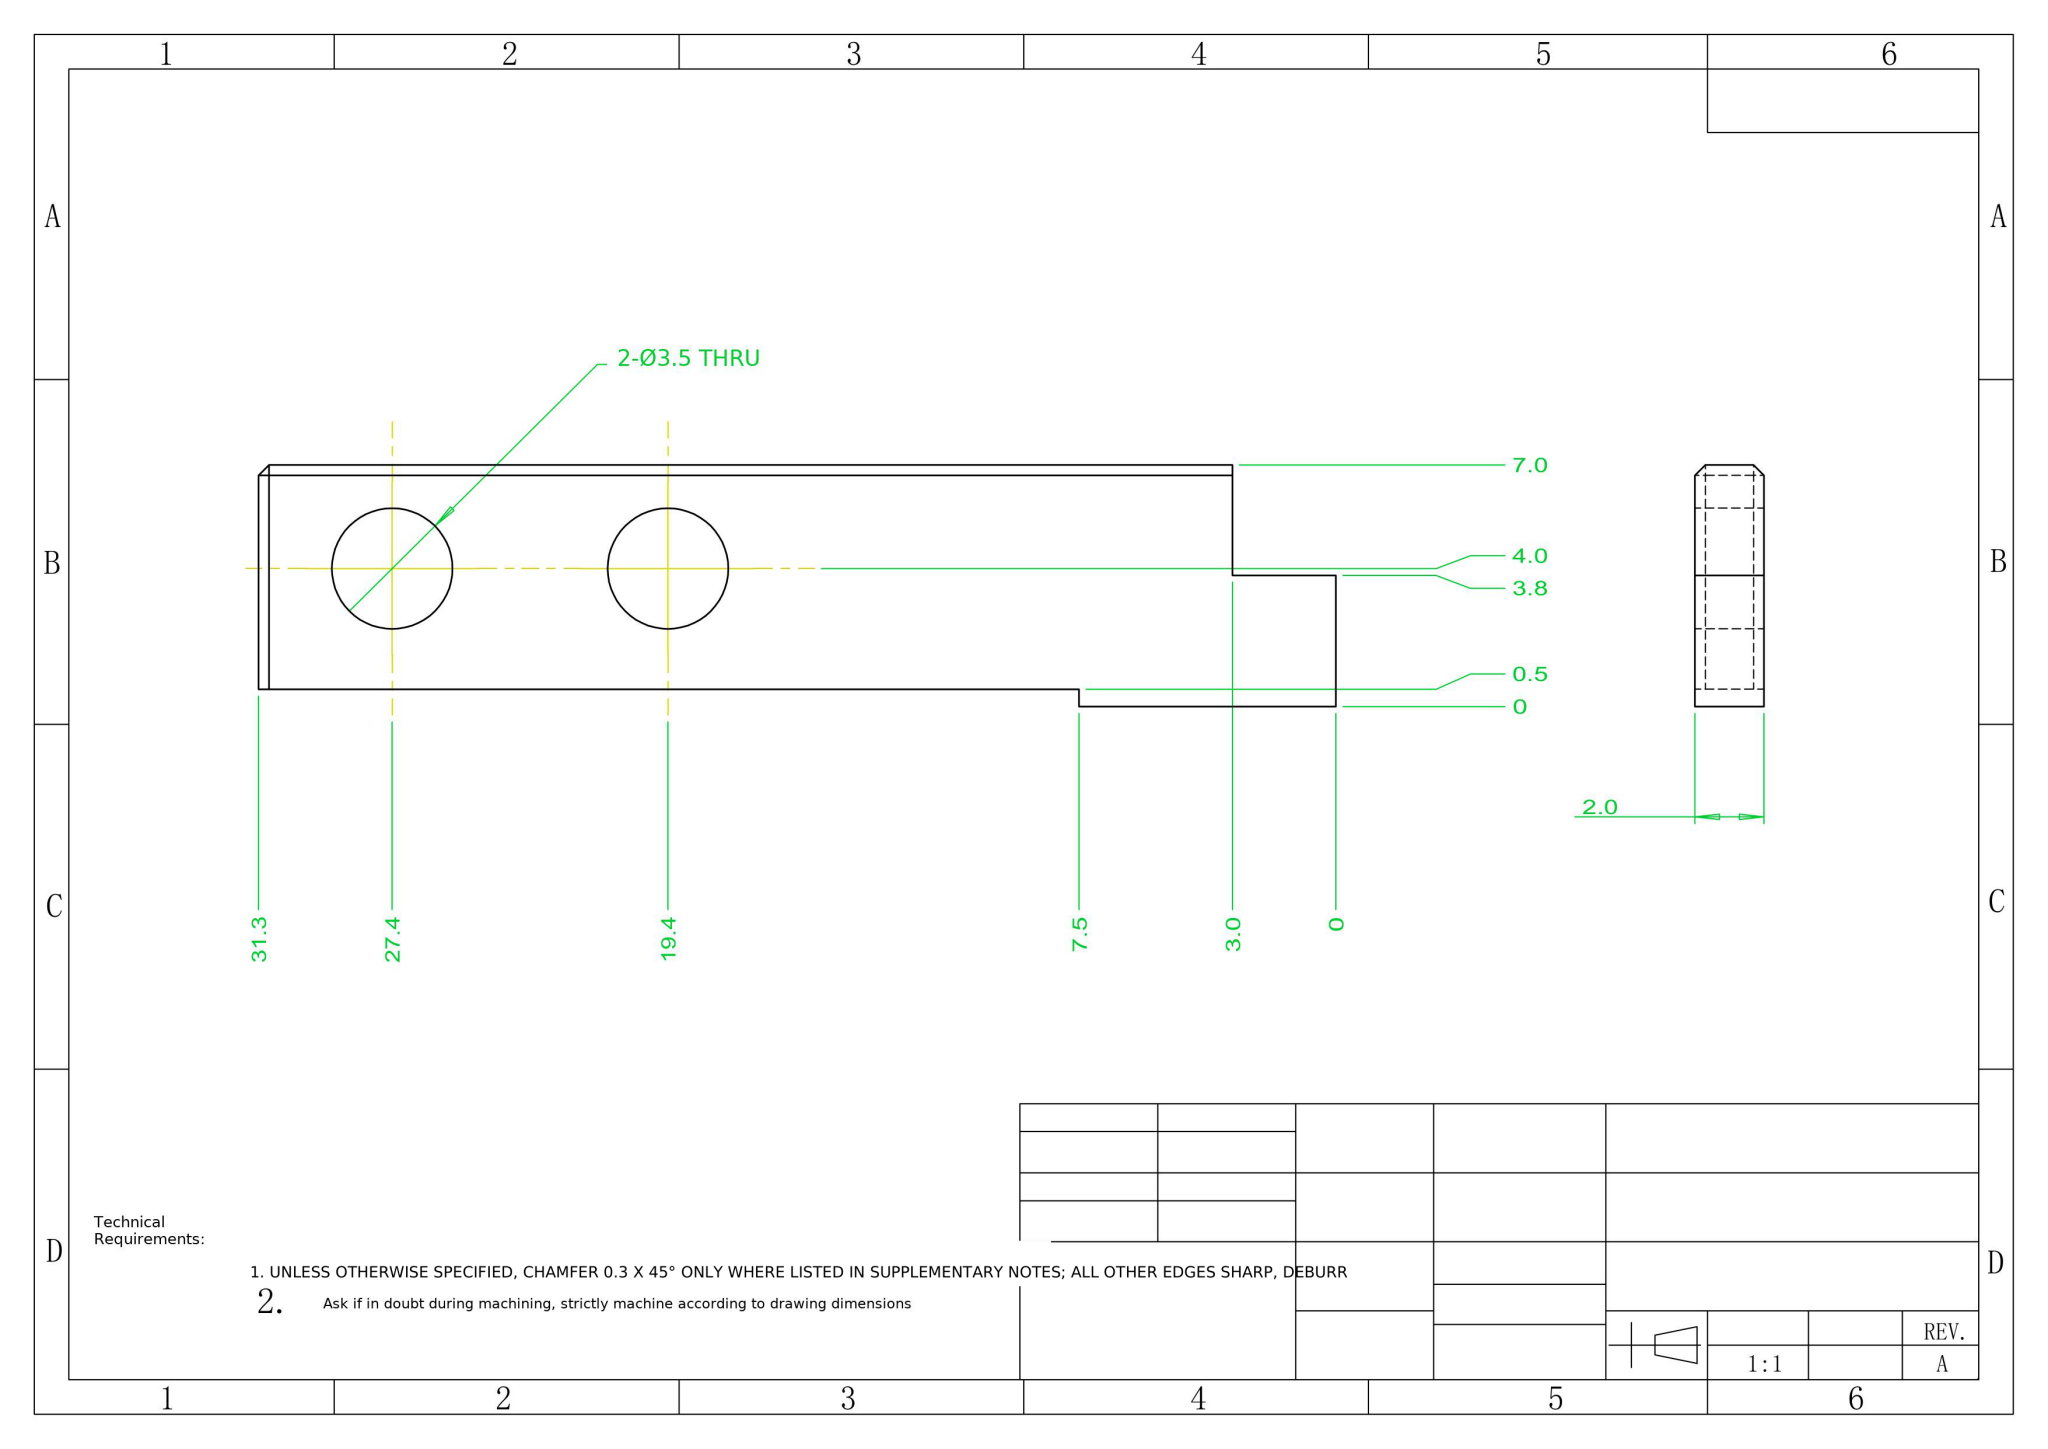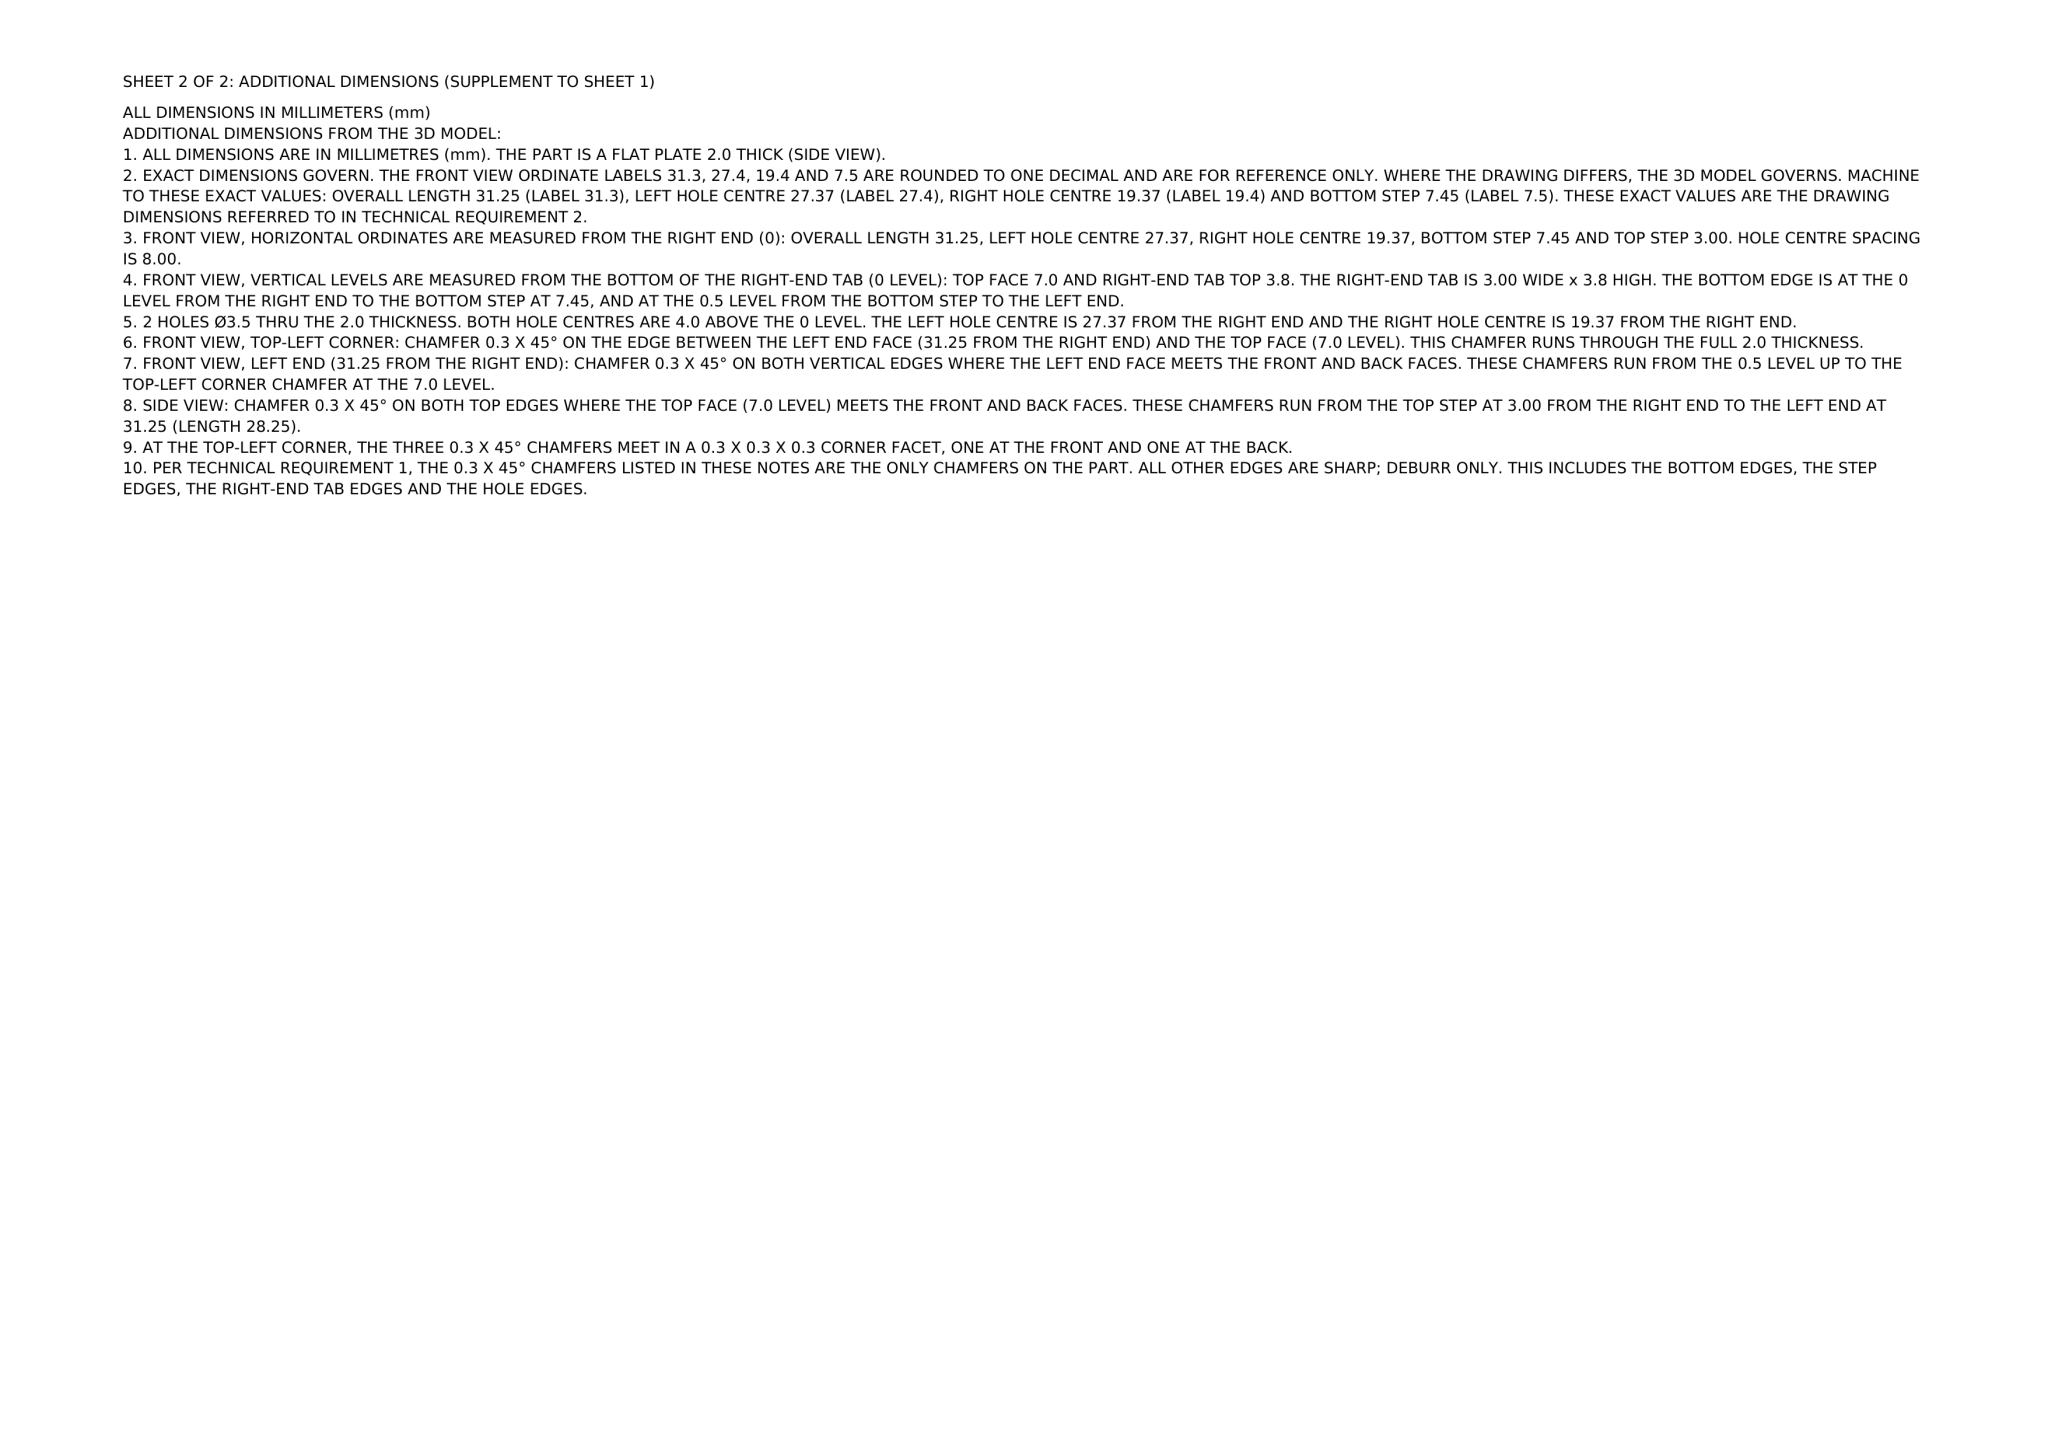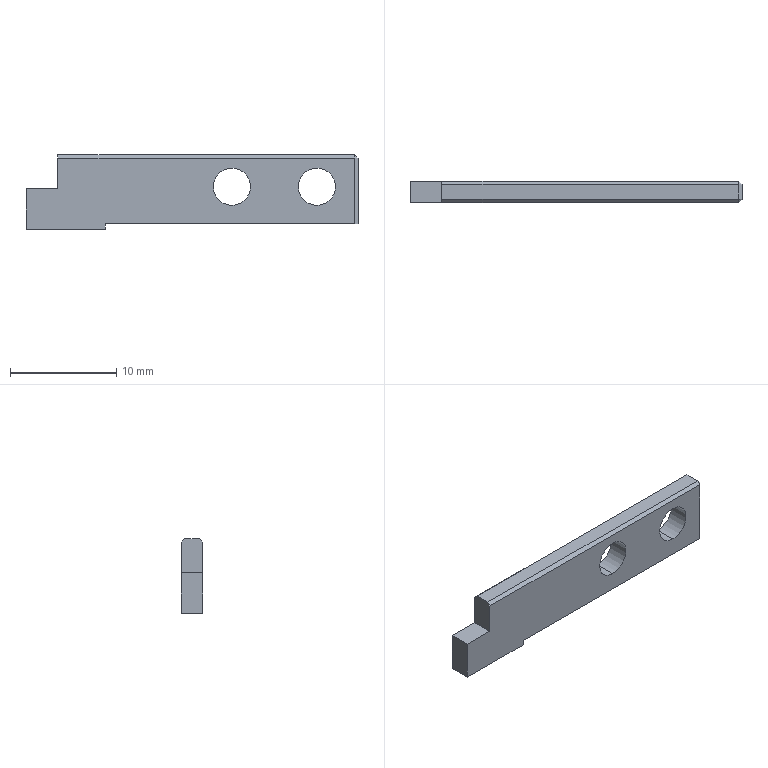Part | NX | mm | Notched Dual-Bore Rail Bracket | 1 solid | 21 faces | box 31.25 x 2 x 7 mm | volume 353 mm3 | plane 17 | cylinder 4 | commonest cylinder face diameters 3.5 x4
STEP:
#1=COLOUR_RGB('',0.502,0.502,1.);
#2=FILL_AREA_STYLE_COLOUR('',#1);
#3=FILL_AREA_STYLE('',(#2));
#4=SURFACE_STYLE_FILL_AREA(#3);
#5=SURFACE_SIDE_STYLE('',(#4));
#6=SURFACE_STYLE_USAGE(.BOTH.,#5);
#7=PRESENTATION_STYLE_ASSIGNMENT((#6));
#8=CARTESIAN_POINT('',(-11.875,0.,-4.75));
#9=VERTEX_POINT('',#8);
#10=CARTESIAN_POINT('',(-11.875,0.,-1.25));
#11=VERTEX_POINT('',#10);
#12=CARTESIAN_POINT('',(-11.875,0.,-3.));
#13=DIRECTION('',(0.,1.,0.));
#14=DIRECTION('',(0.,0.,1.));
#15=AXIS2_PLACEMENT_3D('',#12,#13,#14);
#16=CIRCLE('',#15,1.75);
#17=EDGE_CURVE('',#9,#11,#16,.T.);
#18=ORIENTED_EDGE('',*,*,#17,.F.);
#19=CARTESIAN_POINT('',(-11.875,2.,-4.75));
#20=VERTEX_POINT('',#19);
#21=CARTESIAN_POINT('',(-11.875,0.,-4.75));
#22=DIRECTION('',(0.,1.,0.));
#23=VECTOR('',#22,1000.);
#24=LINE('',#21,#23);
#25=EDGE_CURVE('',#9,#20,#24,.T.);
#26=ORIENTED_EDGE('',*,*,#25,.T.);
#27=CARTESIAN_POINT('',(-11.875,2.,-1.25));
#28=VERTEX_POINT('',#27);
#29=CARTESIAN_POINT('',(-11.875,2.,-3.));
#30=DIRECTION('',(0.,-1.,0.));
#31=DIRECTION('',(0.,0.,1.));
#32=AXIS2_PLACEMENT_3D('',#29,#30,#31);
#33=CIRCLE('',#32,1.75);
#34=EDGE_CURVE('',#28,#20,#33,.T.);
#35=ORIENTED_EDGE('',*,*,#34,.F.);
#36=CARTESIAN_POINT('',(-11.875,0.,-1.25));
#37=DIRECTION('',(0.,1.,0.));
#38=VECTOR('',#37,1000.);
#39=LINE('',#36,#38);
#40=EDGE_CURVE('',#11,#28,#39,.T.);
#41=ORIENTED_EDGE('',*,*,#40,.F.);
#42=EDGE_LOOP('',(#18,#26,#35,#41));
#43=FACE_OUTER_BOUND('',#42,.T.);
#44=CARTESIAN_POINT('',(-11.875,0.,-3.));
#45=DIRECTION('',(0.,1.,0.));
#46=DIRECTION('',(0.,0.,1.));
#47=AXIS2_PLACEMENT_3D('',#44,#45,#46);
#48=CYLINDRICAL_SURFACE('',#47,1.75);
#49=ADVANCED_FACE('',(#43),#48,.F.);
#50=CARTESIAN_POINT('',(-3.875,0.,-4.75));
#51=VERTEX_POINT('',#50);
#52=CARTESIAN_POINT('',(-3.875,0.,-1.25));
#53=VERTEX_POINT('',#52);
#54=CARTESIAN_POINT('',(-3.875,0.,-3.));
#55=DIRECTION('',(0.,1.,0.));
#56=DIRECTION('',(0.,0.,1.));
#57=AXIS2_PLACEMENT_3D('',#54,#55,#56);
#58=CIRCLE('',#57,1.75);
#59=EDGE_CURVE('',#51,#53,#58,.T.);
#60=ORIENTED_EDGE('',*,*,#59,.F.);
#61=CARTESIAN_POINT('',(-3.875,2.,-4.75));
#62=VERTEX_POINT('',#61);
#63=CARTESIAN_POINT('',(-3.875,0.,-4.75));
#64=DIRECTION('',(0.,1.,0.));
#65=VECTOR('',#64,1000.);
#66=LINE('',#63,#65);
#67=EDGE_CURVE('',#51,#62,#66,.T.);
#68=ORIENTED_EDGE('',*,*,#67,.T.);
#69=CARTESIAN_POINT('',(-3.875,2.,-1.25));
#70=VERTEX_POINT('',#69);
#71=CARTESIAN_POINT('',(-3.875,2.,-3.));
#72=DIRECTION('',(0.,-1.,0.));
#73=DIRECTION('',(0.,0.,1.));
#74=AXIS2_PLACEMENT_3D('',#71,#72,#73);
#75=CIRCLE('',#74,1.75);
#76=EDGE_CURVE('',#70,#62,#75,.T.);
#77=ORIENTED_EDGE('',*,*,#76,.F.);
#78=CARTESIAN_POINT('',(-3.875,0.,-1.25));
#79=DIRECTION('',(0.,1.,0.));
#80=VECTOR('',#79,1000.);
#81=LINE('',#78,#80);
#82=EDGE_CURVE('',#53,#70,#81,.T.);
#83=ORIENTED_EDGE('',*,*,#82,.F.);
#84=EDGE_LOOP('',(#60,#68,#77,#83));
#85=FACE_OUTER_BOUND('',#84,.T.);
#86=CARTESIAN_POINT('',(-3.875,0.,-3.));
#87=DIRECTION('',(0.,1.,0.));
#88=DIRECTION('',(0.,0.,1.));
#89=AXIS2_PLACEMENT_3D('',#86,#87,#88);
#90=CYLINDRICAL_SURFACE('',#89,1.75);
#91=ADVANCED_FACE('',(#85),#90,.F.);
#92=CARTESIAN_POINT('',(-0.,0.3,-6.5));
#93=VERTEX_POINT('',#92);
#94=CARTESIAN_POINT('',(-0.3,-0.,-6.5));
#95=VERTEX_POINT('',#94);
#96=CARTESIAN_POINT('',(-0.,0.3,-6.5));
#97=DIRECTION('',(-0.7071,-0.7071,0.));
#98=VECTOR('',#97,1000.);
#99=LINE('',#96,#98);
#100=EDGE_CURVE('',#93,#95,#99,.T.);
#101=ORIENTED_EDGE('',*,*,#100,.F.);
#102=CARTESIAN_POINT('',(0.,0.3,-0.3));
#103=VERTEX_POINT('',#102);
#104=CARTESIAN_POINT('',(0.,0.3,0.));
#105=DIRECTION('',(0.,0.,1.));
#106=VECTOR('',#105,1000.);
#107=LINE('',#104,#106);
#108=EDGE_CURVE('',#93,#103,#107,.T.);
#109=ORIENTED_EDGE('',*,*,#108,.T.);
#110=CARTESIAN_POINT('',(-0.3,-0.,-0.3));
#111=VERTEX_POINT('',#110);
#112=CARTESIAN_POINT('',(-0.,0.3,-0.3));
#113=DIRECTION('',(0.7071,0.7071,0.));
#114=VECTOR('',#113,1000.);
#115=LINE('',#112,#114);
#116=EDGE_CURVE('',#111,#103,#115,.T.);
#117=ORIENTED_EDGE('',*,*,#116,.F.);
#118=CARTESIAN_POINT('',(-0.3,0.,0.));
#119=DIRECTION('',(0.,0.,-1.));
#120=VECTOR('',#119,1000.);
#121=LINE('',#118,#120);
#122=EDGE_CURVE('',#111,#95,#121,.T.);
#123=ORIENTED_EDGE('',*,*,#122,.T.);
#124=EDGE_LOOP('',(#101,#109,#117,#123));
#125=FACE_OUTER_BOUND('',#124,.T.);
#126=CARTESIAN_POINT('',(0.,0.3,0.));
#127=DIRECTION('',(-0.7071,0.7071,0.));
#128=DIRECTION('',(-0.7071,-0.7071,0.));
#129=AXIS2_PLACEMENT_3D('',#126,#127,#128);
#130=PLANE('',#129);
#131=ADVANCED_FACE('',(#125),#130,.F.);
#132=CARTESIAN_POINT('',(-0.,1.7,-6.5));
#133=VERTEX_POINT('',#132);
#134=CARTESIAN_POINT('',(-0.,2.,-6.5));
#135=DIRECTION('',(0.,-1.,0.));
#136=VECTOR('',#135,1000.);
#137=LINE('',#134,#136);
#138=EDGE_CURVE('',#133,#93,#137,.T.);
#139=ORIENTED_EDGE('',*,*,#138,.F.);
#140=CARTESIAN_POINT('',(-0.,1.7,-0.3));
#141=VERTEX_POINT('',#140);
#142=CARTESIAN_POINT('',(-0.,1.7,0.));
#143=DIRECTION('',(-0.,-0.,-1.));
#144=VECTOR('',#143,1000.);
#145=LINE('',#142,#144);
#146=EDGE_CURVE('',#141,#133,#145,.T.);
#147=ORIENTED_EDGE('',*,*,#146,.F.);
#148=CARTESIAN_POINT('',(-0.,2.,-0.3));
#149=DIRECTION('',(0.,1.,0.));
#150=VECTOR('',#149,1000.);
#151=LINE('',#148,#150);
#152=EDGE_CURVE('',#103,#141,#151,.T.);
#153=ORIENTED_EDGE('',*,*,#152,.F.);
#154=ORIENTED_EDGE('',*,*,#108,.F.);
#155=EDGE_LOOP('',(#139,#147,#153,#154));
#156=FACE_OUTER_BOUND('',#155,.T.);
#157=CARTESIAN_POINT('',(0.,2.,0.));
#158=DIRECTION('',(-1.,0.,0.));
#159=DIRECTION('',(0.,0.,1.));
#160=AXIS2_PLACEMENT_3D('',#157,#158,#159);
#161=PLANE('',#160);
#162=ADVANCED_FACE('',(#156),#161,.F.);
#163=ORIENTED_EDGE('',*,*,#146,.T.);
#164=CARTESIAN_POINT('',(-0.3,2.,-6.5));
#165=VERTEX_POINT('',#164);
#166=CARTESIAN_POINT('',(-0.3,2.,-6.5));
#167=DIRECTION('',(-0.7071,0.7071,0.));
#168=VECTOR('',#167,1000.);
#169=LINE('',#166,#168);
#170=EDGE_CURVE('',#133,#165,#169,.T.);
#171=ORIENTED_EDGE('',*,*,#170,.T.);
#172=CARTESIAN_POINT('',(-0.3,2.,-0.3));
#173=VERTEX_POINT('',#172);
#174=CARTESIAN_POINT('',(-0.3,2.,0.));
#175=DIRECTION('',(0.,0.,-1.));
#176=VECTOR('',#175,1000.);
#177=LINE('',#174,#176);
#178=EDGE_CURVE('',#173,#165,#177,.T.);
#179=ORIENTED_EDGE('',*,*,#178,.F.);
#180=CARTESIAN_POINT('',(-0.3,2.,-0.3));
#181=DIRECTION('',(0.7071,-0.7071,0.));
#182=VECTOR('',#181,1000.);
#183=LINE('',#180,#182);
#184=EDGE_CURVE('',#173,#141,#183,.T.);
#185=ORIENTED_EDGE('',*,*,#184,.T.);
#186=EDGE_LOOP('',(#163,#171,#179,#185));
#187=FACE_OUTER_BOUND('',#186,.T.);
#188=CARTESIAN_POINT('',(-0.3,2.,0.));
#189=DIRECTION('',(0.7071,0.7071,-0.));
#190=DIRECTION('',(-0.7071,0.7071,0.));
#191=AXIS2_PLACEMENT_3D('',#188,#189,#190);
#192=PLANE('',#191);
#193=ADVANCED_FACE('',(#187),#192,.T.);
#194=CARTESIAN_POINT('',(-28.25,-0.,-0.3));
#195=VERTEX_POINT('',#194);
#196=CARTESIAN_POINT('',(-28.25,0.3,0.));
#197=VERTEX_POINT('',#196);
#198=CARTESIAN_POINT('',(-28.25,0.3,0.));
#199=DIRECTION('',(0.,0.7071,0.7071));
#200=VECTOR('',#199,1000.);
#201=LINE('',#198,#200);
#202=EDGE_CURVE('',#195,#197,#201,.T.);
#203=ORIENTED_EDGE('',*,*,#202,.F.);
#204=CARTESIAN_POINT('',(0.,0.,-0.3));
#205=DIRECTION('',(1.,0.,0.));
#206=VECTOR('',#205,1000.);
#207=LINE('',#204,#206);
#208=EDGE_CURVE('',#195,#111,#207,.T.);
#209=ORIENTED_EDGE('',*,*,#208,.T.);
#210=CARTESIAN_POINT('',(-0.3,0.3,0.));
#211=VERTEX_POINT('',#210);
#212=CARTESIAN_POINT('',(-0.3,0.3,0.));
#213=DIRECTION('',(0.,-0.7071,-0.7071));
#214=VECTOR('',#213,1000.);
#215=LINE('',#212,#214);
#216=EDGE_CURVE('',#211,#111,#215,.T.);
#217=ORIENTED_EDGE('',*,*,#216,.F.);
#218=CARTESIAN_POINT('',(0.,0.3,0.));
#219=DIRECTION('',(-1.,0.,0.));
#220=VECTOR('',#219,1000.);
#221=LINE('',#218,#220);
#222=EDGE_CURVE('',#211,#197,#221,.T.);
#223=ORIENTED_EDGE('',*,*,#222,.T.);
#224=EDGE_LOOP('',(#203,#209,#217,#223));
#225=FACE_OUTER_BOUND('',#224,.T.);
#226=CARTESIAN_POINT('',(0.,0.3,0.));
#227=DIRECTION('',(-0.,0.7071,-0.7071));
#228=DIRECTION('',(0.,0.7071,0.7071));
#229=AXIS2_PLACEMENT_3D('',#226,#227,#228);
#230=PLANE('',#229);
#231=ADVANCED_FACE('',(#225),#230,.F.);
#232=CARTESIAN_POINT('',(-28.25,1.7,0.));
#233=VERTEX_POINT('',#232);
#234=CARTESIAN_POINT('',(-28.25,2.,0.));
#235=DIRECTION('',(0.,1.,0.));
#236=VECTOR('',#235,1000.);
#237=LINE('',#234,#236);
#238=EDGE_CURVE('',#197,#233,#237,.T.);
#239=ORIENTED_EDGE('',*,*,#238,.F.);
#240=ORIENTED_EDGE('',*,*,#222,.F.);
#241=CARTESIAN_POINT('',(-0.3,1.7,-0.));
#242=VERTEX_POINT('',#241);
#243=CARTESIAN_POINT('',(-0.3,2.,0.));
#244=DIRECTION('',(0.,-1.,0.));
#245=VECTOR('',#244,1000.);
#246=LINE('',#243,#245);
#247=EDGE_CURVE('',#242,#211,#246,.T.);
#248=ORIENTED_EDGE('',*,*,#247,.F.);
#249=CARTESIAN_POINT('',(-0.,1.7,-0.));
#250=DIRECTION('',(1.,-0.,-0.));
#251=VECTOR('',#250,1000.);
#252=LINE('',#249,#251);
#253=EDGE_CURVE('',#233,#242,#252,.T.);
#254=ORIENTED_EDGE('',*,*,#253,.F.);
#255=EDGE_LOOP('',(#239,#240,#248,#254));
#256=FACE_OUTER_BOUND('',#255,.T.);
#257=CARTESIAN_POINT('',(0.,2.,0.));
#258=DIRECTION('',(-0.,0.,-1.));
#259=DIRECTION('',(-1.,0.,0.));
#260=AXIS2_PLACEMENT_3D('',#257,#258,#259);
#261=PLANE('',#260);
#262=ADVANCED_FACE('',(#256),#261,.F.);
#263=CARTESIAN_POINT('',(-28.25,2.,-0.3));
#264=VERTEX_POINT('',#263);
#265=CARTESIAN_POINT('',(0.,2.,-0.3));
#266=DIRECTION('',(1.,0.,0.));
#267=VECTOR('',#266,1000.);
#268=LINE('',#265,#267);
#269=EDGE_CURVE('',#264,#173,#268,.T.);
#270=ORIENTED_EDGE('',*,*,#269,.F.);
#271=CARTESIAN_POINT('',(-28.25,2.,-0.3));
#272=DIRECTION('',(0.,-0.7071,0.7071));
#273=VECTOR('',#272,1000.);
#274=LINE('',#271,#273);
#275=EDGE_CURVE('',#264,#233,#274,.T.);
#276=ORIENTED_EDGE('',*,*,#275,.T.);
#277=ORIENTED_EDGE('',*,*,#253,.T.);
#278=CARTESIAN_POINT('',(-0.3,2.,-0.3));
#279=DIRECTION('',(0.,0.7071,-0.7071));
#280=VECTOR('',#279,1000.);
#281=LINE('',#278,#280);
#282=EDGE_CURVE('',#242,#173,#281,.T.);
#283=ORIENTED_EDGE('',*,*,#282,.T.);
#284=EDGE_LOOP('',(#270,#276,#277,#283));
#285=FACE_OUTER_BOUND('',#284,.T.);
#286=CARTESIAN_POINT('',(-0.,2.,-0.3));
#287=DIRECTION('',(0.,0.7071,0.7071));
#288=DIRECTION('',(0.,-0.7071,0.7071));
#289=AXIS2_PLACEMENT_3D('',#286,#287,#288);
#290=PLANE('',#289);
#291=ADVANCED_FACE('',(#285),#290,.T.);
#292=CARTESIAN_POINT('',(-31.25,2.,-7.));
#293=VERTEX_POINT('',#292);
#294=CARTESIAN_POINT('',(-31.25,0.,-7.));
#295=VERTEX_POINT('',#294);
#296=CARTESIAN_POINT('',(-31.25,2.,-7.));
#297=DIRECTION('',(0.,-1.,0.));
#298=VECTOR('',#297,1000.);
#299=LINE('',#296,#298);
#300=EDGE_CURVE('',#293,#295,#299,.T.);
#301=ORIENTED_EDGE('',*,*,#300,.T.);
#302=CARTESIAN_POINT('',(-31.25,0.,-3.2));
#303=VERTEX_POINT('',#302);
#304=CARTESIAN_POINT('',(-31.25,0.,0.));
#305=DIRECTION('',(0.,0.,1.));
#306=VECTOR('',#305,1000.);
#307=LINE('',#304,#306);
#308=EDGE_CURVE('',#295,#303,#307,.T.);
#309=ORIENTED_EDGE('',*,*,#308,.T.);
#310=CARTESIAN_POINT('',(-31.25,2.,-3.2));
#311=VERTEX_POINT('',#310);
#312=CARTESIAN_POINT('',(-31.25,5.153,-3.2));
#313=DIRECTION('',(0.,-1.,0.));
#314=VECTOR('',#313,1000.);
#315=LINE('',#312,#314);
#316=EDGE_CURVE('',#311,#303,#315,.T.);
#317=ORIENTED_EDGE('',*,*,#316,.F.);
#318=CARTESIAN_POINT('',(-31.25,2.,0.));
#319=DIRECTION('',(0.,0.,1.));
#320=VECTOR('',#319,1000.);
#321=LINE('',#318,#320);
#322=EDGE_CURVE('',#293,#311,#321,.T.);
#323=ORIENTED_EDGE('',*,*,#322,.F.);
#324=EDGE_LOOP('',(#301,#309,#317,#323));
#325=FACE_OUTER_BOUND('',#324,.T.);
#326=CARTESIAN_POINT('',(-31.25,2.,0.));
#327=DIRECTION('',(1.,0.,0.));
#328=DIRECTION('',(0.,0.,-1.));
#329=AXIS2_PLACEMENT_3D('',#326,#327,#328);
#330=PLANE('',#329);
#331=ADVANCED_FACE('',(#325),#330,.F.);
#332=CARTESIAN_POINT('',(-23.8,2.,-7.));
#333=VERTEX_POINT('',#332);
#334=CARTESIAN_POINT('',(-23.8,2.,-6.5));
#335=VERTEX_POINT('',#334);
#336=CARTESIAN_POINT('',(-23.8,2.,0.));
#337=DIRECTION('',(0.,0.,1.));
#338=VECTOR('',#337,1000.);
#339=LINE('',#336,#338);
#340=EDGE_CURVE('',#333,#335,#339,.T.);
#341=ORIENTED_EDGE('',*,*,#340,.F.);
#342=CARTESIAN_POINT('',(0.,2.,-7.));
#343=DIRECTION('',(-1.,0.,0.));
#344=VECTOR('',#343,1000.);
#345=LINE('',#342,#344);
#346=EDGE_CURVE('',#333,#293,#345,.T.);
#347=ORIENTED_EDGE('',*,*,#346,.T.);
#348=ORIENTED_EDGE('',*,*,#322,.T.);
#349=CARTESIAN_POINT('',(-28.25,2.,-3.2));
#350=VERTEX_POINT('',#349);
#351=CARTESIAN_POINT('',(0.,2.,-3.2));
#352=DIRECTION('',(-1.,0.,0.));
#353=VECTOR('',#352,1000.);
#354=LINE('',#351,#353);
#355=EDGE_CURVE('',#350,#311,#354,.T.);
#356=ORIENTED_EDGE('',*,*,#355,.F.);
#357=CARTESIAN_POINT('',(-28.25,2.,0.));
#358=DIRECTION('',(0.,0.,1.));
#359=VECTOR('',#358,1000.);
#360=LINE('',#357,#359);
#361=EDGE_CURVE('',#350,#264,#360,.T.);
#362=ORIENTED_EDGE('',*,*,#361,.T.);
#363=ORIENTED_EDGE('',*,*,#269,.T.);
#364=ORIENTED_EDGE('',*,*,#178,.T.);
#365=CARTESIAN_POINT('',(-0.,2.,-6.5));
#366=DIRECTION('',(-1.,0.,0.));
#367=VECTOR('',#366,1000.);
#368=LINE('',#365,#367);
#369=EDGE_CURVE('',#165,#335,#368,.T.);
#370=ORIENTED_EDGE('',*,*,#369,.T.);
#371=EDGE_LOOP('',(#341,#347,#348,#356,#362,#363,#364,#370));
#372=FACE_OUTER_BOUND('',#371,.T.);
#373=ORIENTED_EDGE('',*,*,#34,.T.);
#374=CARTESIAN_POINT('',(-11.875,2.,-3.));
#375=DIRECTION('',(0.,-1.,0.));
#376=DIRECTION('',(0.,0.,1.));
#377=AXIS2_PLACEMENT_3D('',#374,#375,#376);
#378=CIRCLE('',#377,1.75);
#379=EDGE_CURVE('',#20,#28,#378,.T.);
#380=ORIENTED_EDGE('',*,*,#379,.T.);
#381=EDGE_LOOP('',(#373,#380));
#382=FACE_BOUND('',#381,.T.);
#383=ORIENTED_EDGE('',*,*,#76,.T.);
#384=CARTESIAN_POINT('',(-3.875,2.,-3.));
#385=DIRECTION('',(0.,-1.,0.));
#386=DIRECTION('',(0.,0.,1.));
#387=AXIS2_PLACEMENT_3D('',#384,#385,#386);
#388=CIRCLE('',#387,1.75);
#389=EDGE_CURVE('',#62,#70,#388,.T.);
#390=ORIENTED_EDGE('',*,*,#389,.T.);
#391=EDGE_LOOP('',(#383,#390));
#392=FACE_BOUND('',#391,.T.);
#393=CARTESIAN_POINT('',(0.,2.,0.));
#394=DIRECTION('',(0.,1.,0.));
#395=DIRECTION('',(0.,0.,1.));
#396=AXIS2_PLACEMENT_3D('',#393,#394,#395);
#397=PLANE('',#396);
#398=ADVANCED_FACE('',(#372,#382,#392),#397,.T.);
#399=ORIENTED_EDGE('',*,*,#25,.F.);
#400=CARTESIAN_POINT('',(-11.875,0.,-3.));
#401=DIRECTION('',(0.,1.,0.));
#402=DIRECTION('',(0.,0.,1.));
#403=AXIS2_PLACEMENT_3D('',#400,#401,#402);
#404=CIRCLE('',#403,1.75);
#405=EDGE_CURVE('',#11,#9,#404,.T.);
#406=ORIENTED_EDGE('',*,*,#405,.F.);
#407=ORIENTED_EDGE('',*,*,#40,.T.);
#408=ORIENTED_EDGE('',*,*,#379,.F.);
#409=EDGE_LOOP('',(#399,#406,#407,#408));
#410=FACE_OUTER_BOUND('',#409,.T.);
#411=CARTESIAN_POINT('',(-11.875,0.,-3.));
#412=DIRECTION('',(0.,1.,0.));
#413=DIRECTION('',(0.,0.,1.));
#414=AXIS2_PLACEMENT_3D('',#411,#412,#413);
#415=CYLINDRICAL_SURFACE('',#414,1.75);
#416=ADVANCED_FACE('',(#410),#415,.F.);
#417=ORIENTED_EDGE('',*,*,#67,.F.);
#418=CARTESIAN_POINT('',(-3.875,0.,-3.));
#419=DIRECTION('',(0.,1.,0.));
#420=DIRECTION('',(0.,0.,1.));
#421=AXIS2_PLACEMENT_3D('',#418,#419,#420);
#422=CIRCLE('',#421,1.75);
#423=EDGE_CURVE('',#53,#51,#422,.T.);
#424=ORIENTED_EDGE('',*,*,#423,.F.);
#425=ORIENTED_EDGE('',*,*,#82,.T.);
#426=ORIENTED_EDGE('',*,*,#389,.F.);
#427=EDGE_LOOP('',(#417,#424,#425,#426));
#428=FACE_OUTER_BOUND('',#427,.T.);
#429=CARTESIAN_POINT('',(-3.875,0.,-3.));
#430=DIRECTION('',(0.,1.,0.));
#431=DIRECTION('',(0.,0.,1.));
#432=AXIS2_PLACEMENT_3D('',#429,#430,#431);
#433=CYLINDRICAL_SURFACE('',#432,1.75);
#434=ADVANCED_FACE('',(#428),#433,.F.);
#435=CARTESIAN_POINT('',(-23.8,0.,-7.));
#436=VERTEX_POINT('',#435);
#437=CARTESIAN_POINT('',(-0.,0.,-7.));
#438=DIRECTION('',(1.,0.,-0.));
#439=VECTOR('',#438,1000.);
#440=LINE('',#437,#439);
#441=EDGE_CURVE('',#295,#436,#440,.T.);
#442=ORIENTED_EDGE('',*,*,#441,.T.);
#443=CARTESIAN_POINT('',(-23.8,0.,-6.5));
#444=VERTEX_POINT('',#443);
#445=CARTESIAN_POINT('',(-23.8,0.,0.));
#446=DIRECTION('',(0.,0.,1.));
#447=VECTOR('',#446,1000.);
#448=LINE('',#445,#447);
#449=EDGE_CURVE('',#436,#444,#448,.T.);
#450=ORIENTED_EDGE('',*,*,#449,.T.);
#451=CARTESIAN_POINT('',(-0.,0.,-6.5));
#452=DIRECTION('',(-1.,0.,0.));
#453=VECTOR('',#452,1000.);
#454=LINE('',#451,#453);
#455=EDGE_CURVE('',#95,#444,#454,.T.);
#456=ORIENTED_EDGE('',*,*,#455,.F.);
#457=ORIENTED_EDGE('',*,*,#122,.F.);
#458=ORIENTED_EDGE('',*,*,#208,.F.);
#459=CARTESIAN_POINT('',(-28.25,0.,-3.2));
#460=VERTEX_POINT('',#459);
#461=CARTESIAN_POINT('',(-28.25,0.,0.));
#462=DIRECTION('',(0.,0.,1.));
#463=VECTOR('',#462,1000.);
#464=LINE('',#461,#463);
#465=EDGE_CURVE('',#460,#195,#464,.T.);
#466=ORIENTED_EDGE('',*,*,#465,.F.);
#467=CARTESIAN_POINT('',(0.,0.,-3.2));
#468=DIRECTION('',(-1.,0.,0.));
#469=VECTOR('',#468,1000.);
#470=LINE('',#467,#469);
#471=EDGE_CURVE('',#460,#303,#470,.T.);
#472=ORIENTED_EDGE('',*,*,#471,.T.);
#473=ORIENTED_EDGE('',*,*,#308,.F.);
#474=EDGE_LOOP('',(#442,#450,#456,#457,#458,#466,#472,#473));
#475=FACE_OUTER_BOUND('',#474,.T.);
#476=ORIENTED_EDGE('',*,*,#405,.T.);
#477=ORIENTED_EDGE('',*,*,#17,.T.);
#478=EDGE_LOOP('',(#476,#477));
#479=FACE_BOUND('',#478,.T.);
#480=ORIENTED_EDGE('',*,*,#423,.T.);
#481=ORIENTED_EDGE('',*,*,#59,.T.);
#482=EDGE_LOOP('',(#480,#481));
#483=FACE_BOUND('',#482,.T.);
#484=CARTESIAN_POINT('',(0.,0.,0.));
#485=DIRECTION('',(0.,1.,0.));
#486=DIRECTION('',(0.,0.,1.));
#487=AXIS2_PLACEMENT_3D('',#484,#485,#486);
#488=PLANE('',#487);
#489=ADVANCED_FACE('',(#475,#479,#483),#488,.F.);
#490=ORIENTED_EDGE('',*,*,#184,.F.);
#491=ORIENTED_EDGE('',*,*,#282,.F.);
#492=CARTESIAN_POINT('',(-0.15,1.7,-0.15));
#493=DIRECTION('',(0.7071,0.,-0.7071));
#494=VECTOR('',#493,1000.);
#495=LINE('',#492,#494);
#496=EDGE_CURVE('',#242,#141,#495,.T.);
#497=ORIENTED_EDGE('',*,*,#496,.T.);
#498=EDGE_LOOP('',(#490,#491,#497));
#499=FACE_OUTER_BOUND('',#498,.T.);
#500=CARTESIAN_POINT('',(-0.3,2.,-0.3));
#501=DIRECTION('',(0.5774,0.5774,0.5774));
#502=DIRECTION('',(0.7071,0.,-0.7071));
#503=AXIS2_PLACEMENT_3D('',#500,#501,#502);
#504=PLANE('',#503);
#505=ADVANCED_FACE('',(#499),#504,.T.);
#506=ORIENTED_EDGE('',*,*,#346,.F.);
#507=CARTESIAN_POINT('',(-23.8,-1.124,-7.));
#508=DIRECTION('',(0.,1.,0.));
#509=VECTOR('',#508,1000.);
#510=LINE('',#507,#509);
#511=EDGE_CURVE('',#436,#333,#510,.T.);
#512=ORIENTED_EDGE('',*,*,#511,.F.);
#513=ORIENTED_EDGE('',*,*,#441,.F.);
#514=ORIENTED_EDGE('',*,*,#300,.F.);
#515=EDGE_LOOP('',(#506,#512,#513,#514));
#516=FACE_OUTER_BOUND('',#515,.T.);
#517=CARTESIAN_POINT('',(0.,2.,-7.));
#518=DIRECTION('',(0.,0.,1.));
#519=DIRECTION('',(1.,0.,-0.));
#520=AXIS2_PLACEMENT_3D('',#517,#518,#519);
#521=PLANE('',#520);
#522=ADVANCED_FACE('',(#516),#521,.F.);
#523=ORIENTED_EDGE('',*,*,#152,.T.);
#524=ORIENTED_EDGE('',*,*,#496,.F.);
#525=ORIENTED_EDGE('',*,*,#247,.T.);
#526=CARTESIAN_POINT('',(-0.,0.3,-0.3));
#527=DIRECTION('',(-0.7071,0.,0.7071));
#528=VECTOR('',#527,1000.);
#529=LINE('',#526,#528);
#530=EDGE_CURVE('',#103,#211,#529,.T.);
#531=ORIENTED_EDGE('',*,*,#530,.F.);
#532=EDGE_LOOP('',(#523,#524,#525,#531));
#533=FACE_OUTER_BOUND('',#532,.T.);
#534=CARTESIAN_POINT('',(-0.,2.,-0.3));
#535=DIRECTION('',(-0.7071,0.,-0.7071));
#536=DIRECTION('',(-0.7071,0.,0.7071));
#537=AXIS2_PLACEMENT_3D('',#534,#535,#536);
#538=PLANE('',#537);
#539=ADVANCED_FACE('',(#533),#538,.F.);
#540=ORIENTED_EDGE('',*,*,#116,.T.);
#541=ORIENTED_EDGE('',*,*,#530,.T.);
#542=ORIENTED_EDGE('',*,*,#216,.T.);
#543=EDGE_LOOP('',(#540,#541,#542));
#544=FACE_OUTER_BOUND('',#543,.T.);
#545=CARTESIAN_POINT('',(-0.3,0.3,0.));
#546=DIRECTION('',(0.5774,-0.5774,0.5774));
#547=DIRECTION('',(0.7071,0.,-0.7071));
#548=AXIS2_PLACEMENT_3D('',#545,#546,#547);
#549=PLANE('',#548);
#550=ADVANCED_FACE('',(#544),#549,.T.);
#551=CARTESIAN_POINT('',(-28.25,5.153,-3.2));
#552=DIRECTION('',(0.,-1.,0.));
#553=VECTOR('',#552,1000.);
#554=LINE('',#551,#553);
#555=EDGE_CURVE('',#350,#460,#554,.T.);
#556=ORIENTED_EDGE('',*,*,#555,.F.);
#557=ORIENTED_EDGE('',*,*,#355,.T.);
#558=ORIENTED_EDGE('',*,*,#316,.T.);
#559=ORIENTED_EDGE('',*,*,#471,.F.);
#560=EDGE_LOOP('',(#556,#557,#558,#559));
#561=FACE_OUTER_BOUND('',#560,.T.);
#562=CARTESIAN_POINT('',(-28.25,5.153,-3.2));
#563=DIRECTION('',(0.,-0.,-1.));
#564=DIRECTION('',(0.,1.,-0.));
#565=AXIS2_PLACEMENT_3D('',#562,#563,#564);
#566=PLANE('',#565);
#567=ADVANCED_FACE('',(#561),#566,.F.);
#568=ORIENTED_EDGE('',*,*,#465,.T.);
#569=ORIENTED_EDGE('',*,*,#202,.T.);
#570=ORIENTED_EDGE('',*,*,#238,.T.);
#571=ORIENTED_EDGE('',*,*,#275,.F.);
#572=ORIENTED_EDGE('',*,*,#361,.F.);
#573=ORIENTED_EDGE('',*,*,#555,.T.);
#574=EDGE_LOOP('',(#568,#569,#570,#571,#572,#573));
#575=FACE_OUTER_BOUND('',#574,.T.);
#576=CARTESIAN_POINT('',(-28.25,0.,0.));
#577=DIRECTION('',(-1.,0.,0.));
#578=DIRECTION('',(0.,0.,1.));
#579=AXIS2_PLACEMENT_3D('',#576,#577,#578);
#580=PLANE('',#579);
#581=ADVANCED_FACE('',(#575),#580,.T.);
#582=ORIENTED_EDGE('',*,*,#511,.T.);
#583=ORIENTED_EDGE('',*,*,#340,.T.);
#584=CARTESIAN_POINT('',(-23.8,0.,-6.5));
#585=DIRECTION('',(0.,1.,0.));
#586=VECTOR('',#585,1000.);
#587=LINE('',#584,#586);
#588=EDGE_CURVE('',#444,#335,#587,.T.);
#589=ORIENTED_EDGE('',*,*,#588,.F.);
#590=ORIENTED_EDGE('',*,*,#449,.F.);
#591=EDGE_LOOP('',(#582,#583,#589,#590));
#592=FACE_OUTER_BOUND('',#591,.T.);
#593=CARTESIAN_POINT('',(-23.8,-1.124,-6.5));
#594=DIRECTION('',(-1.,0.,0.));
#595=DIRECTION('',(0.,0.,1.));
#596=AXIS2_PLACEMENT_3D('',#593,#594,#595);
#597=PLANE('',#596);
#598=ADVANCED_FACE('',(#592),#597,.F.);
#599=ORIENTED_EDGE('',*,*,#455,.T.);
#600=ORIENTED_EDGE('',*,*,#588,.T.);
#601=ORIENTED_EDGE('',*,*,#369,.F.);
#602=ORIENTED_EDGE('',*,*,#170,.F.);
#603=ORIENTED_EDGE('',*,*,#138,.T.);
#604=ORIENTED_EDGE('',*,*,#100,.T.);
#605=EDGE_LOOP('',(#599,#600,#601,#602,#603,#604));
#606=FACE_OUTER_BOUND('',#605,.T.);
#607=CARTESIAN_POINT('',(-0.,0.,-6.5));
#608=DIRECTION('',(-0.,0.,-1.));
#609=DIRECTION('',(-1.,0.,0.));
#610=AXIS2_PLACEMENT_3D('',#607,#608,#609);
#611=PLANE('',#610);
#612=ADVANCED_FACE('',(#606),#611,.T.);
#613=CLOSED_SHELL('',(#49,#91,#131,#162,#193,#231,#262,#291,#331,#398,#416,#434,#489,#505,#522,#539,#550,#567,#581,#598,#612));
#614=MANIFOLD_SOLID_BREP('',#613);
#615=CARTESIAN_POINT('',(0.,0.,0.));
#616=DIRECTION('',(0.,0.,1.));
#617=DIRECTION('',(1.,0.,0.));
#618=AXIS2_PLACEMENT_3D('',#615,#616,#617);
#619=(LENGTH_UNIT()NAMED_UNIT(*)SI_UNIT(.MILLI.,.METRE.));
#620=UNCERTAINTY_MEASURE_WITH_UNIT(LENGTH_MEASURE(0.00001),#619,'','');
#621=(NAMED_UNIT(*)PLANE_ANGLE_UNIT()SI_UNIT($,.RADIAN.));
#622=(NAMED_UNIT(*)SI_UNIT($,.STERADIAN.)SOLID_ANGLE_UNIT());
#623=(GEOMETRIC_REPRESENTATION_CONTEXT(3)GLOBAL_UNCERTAINTY_ASSIGNED_CONTEXT((#620))GLOBAL_UNIT_ASSIGNED_CONTEXT((#619,#621,#622))REPRESENTATION_CONTEXT('',''));
#624=ADVANCED_BREP_SHAPE_REPRESENTATION('',(#614,#618),#623);
#625=STYLED_ITEM('',(#7),#624);
#626=(LENGTH_UNIT()NAMED_UNIT(*)SI_UNIT(.MILLI.,.METRE.));
#627=UNCERTAINTY_MEASURE_WITH_UNIT(LENGTH_MEASURE(0.00001),#626,'','');
#628=(NAMED_UNIT(*)PLANE_ANGLE_UNIT()SI_UNIT($,.RADIAN.));
#629=(NAMED_UNIT(*)SI_UNIT($,.STERADIAN.)SOLID_ANGLE_UNIT());
#630=(GEOMETRIC_REPRESENTATION_CONTEXT(3)GLOBAL_UNCERTAINTY_ASSIGNED_CONTEXT((#627))GLOBAL_UNIT_ASSIGNED_CONTEXT((#626,#628,#629))REPRESENTATION_CONTEXT('',''));
#631=MECHANICAL_DESIGN_GEOMETRIC_PRESENTATION_REPRESENTATION('',(#625),#630);
#632=PRESENTATION_LAYER_ASSIGNMENT('','',(#625));
#633=COLOUR_RGB('',0.502,0.502,1.);
#634=FILL_AREA_STYLE_COLOUR('',#633);
#635=FILL_AREA_STYLE('',(#634));
#636=SURFACE_STYLE_FILL_AREA(#635);
#637=SURFACE_SIDE_STYLE('',(#636));
#638=SURFACE_STYLE_USAGE(.BOTH.,#637);
#639=PRESENTATION_STYLE_ASSIGNMENT((#638));
#640=STYLED_ITEM('',(#639),#614);
#641=(LENGTH_UNIT()NAMED_UNIT(*)SI_UNIT(.MILLI.,.METRE.));
#642=UNCERTAINTY_MEASURE_WITH_UNIT(LENGTH_MEASURE(0.00001),#641,'','');
#643=(NAMED_UNIT(*)PLANE_ANGLE_UNIT()SI_UNIT($,.RADIAN.));
#644=(NAMED_UNIT(*)SI_UNIT($,.STERADIAN.)SOLID_ANGLE_UNIT());
#645=(GEOMETRIC_REPRESENTATION_CONTEXT(3)GLOBAL_UNCERTAINTY_ASSIGNED_CONTEXT((#642))GLOBAL_UNIT_ASSIGNED_CONTEXT((#641,#643,#644))REPRESENTATION_CONTEXT('',''));
#646=MECHANICAL_DESIGN_GEOMETRIC_PRESENTATION_REPRESENTATION('',(#640),#645);
#647=PRESENTATION_LAYER_ASSIGNMENT('','',(#640));